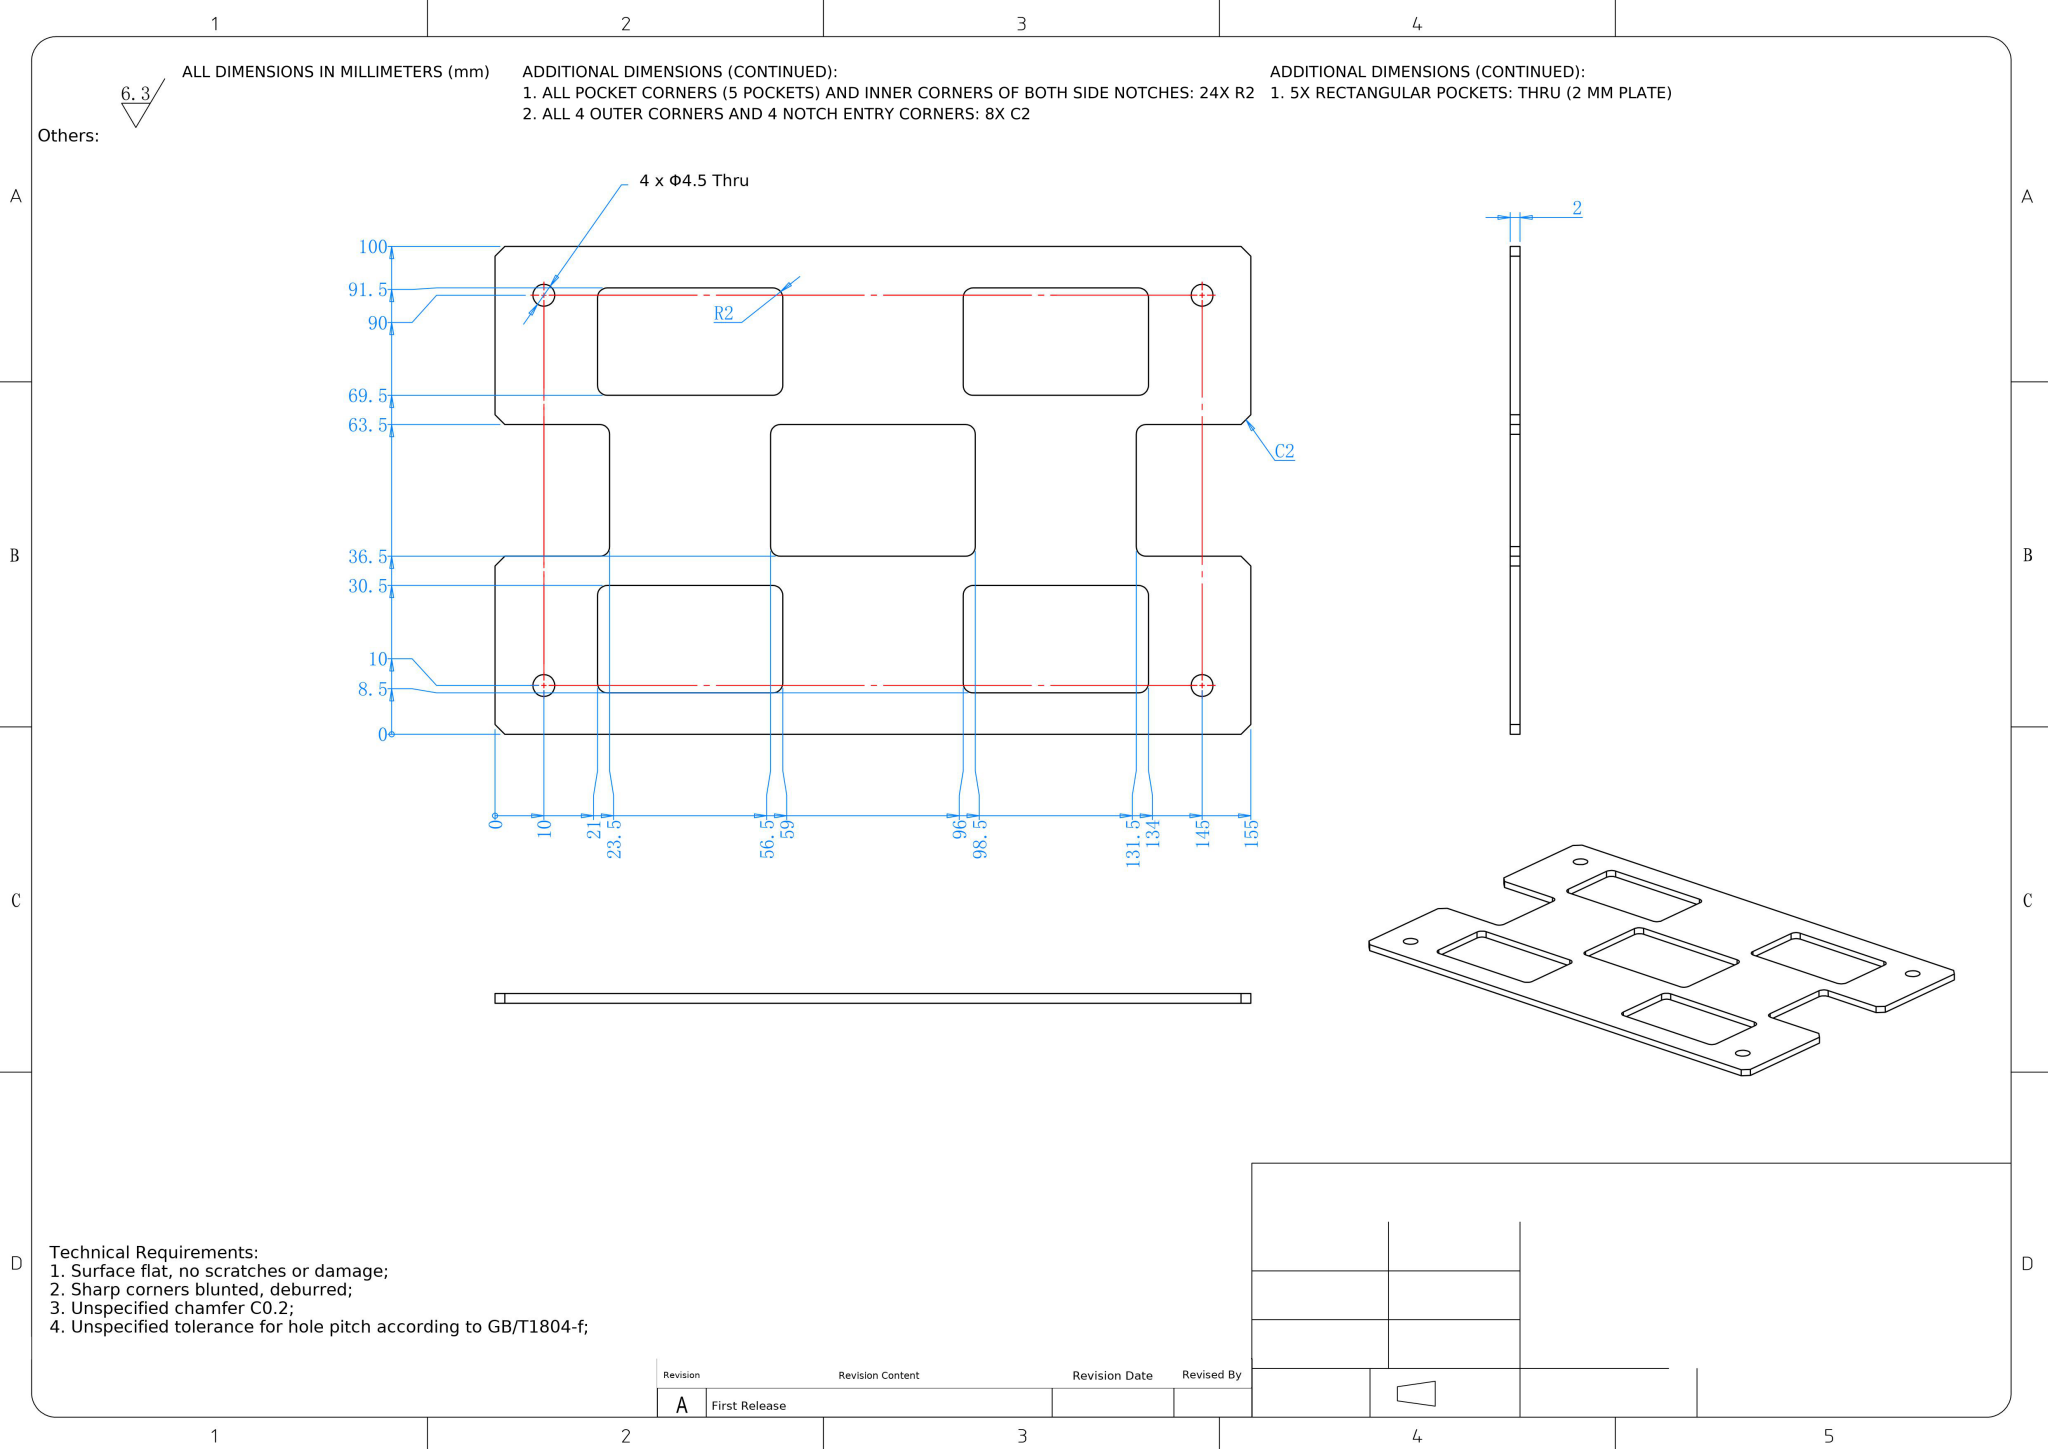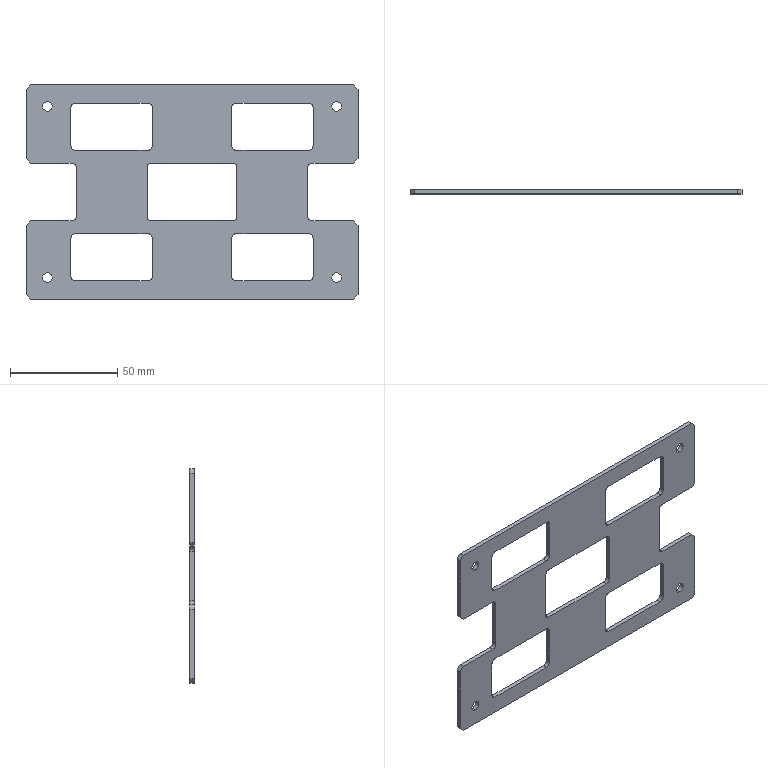Part | NX | mm | 1 solid | 74 faces | box 155 x 2 x 100 mm | volume 19388 mm3 | plane 42 | cylinder 32 | commonest cylinder face diameters 4 x24 4.5 x8